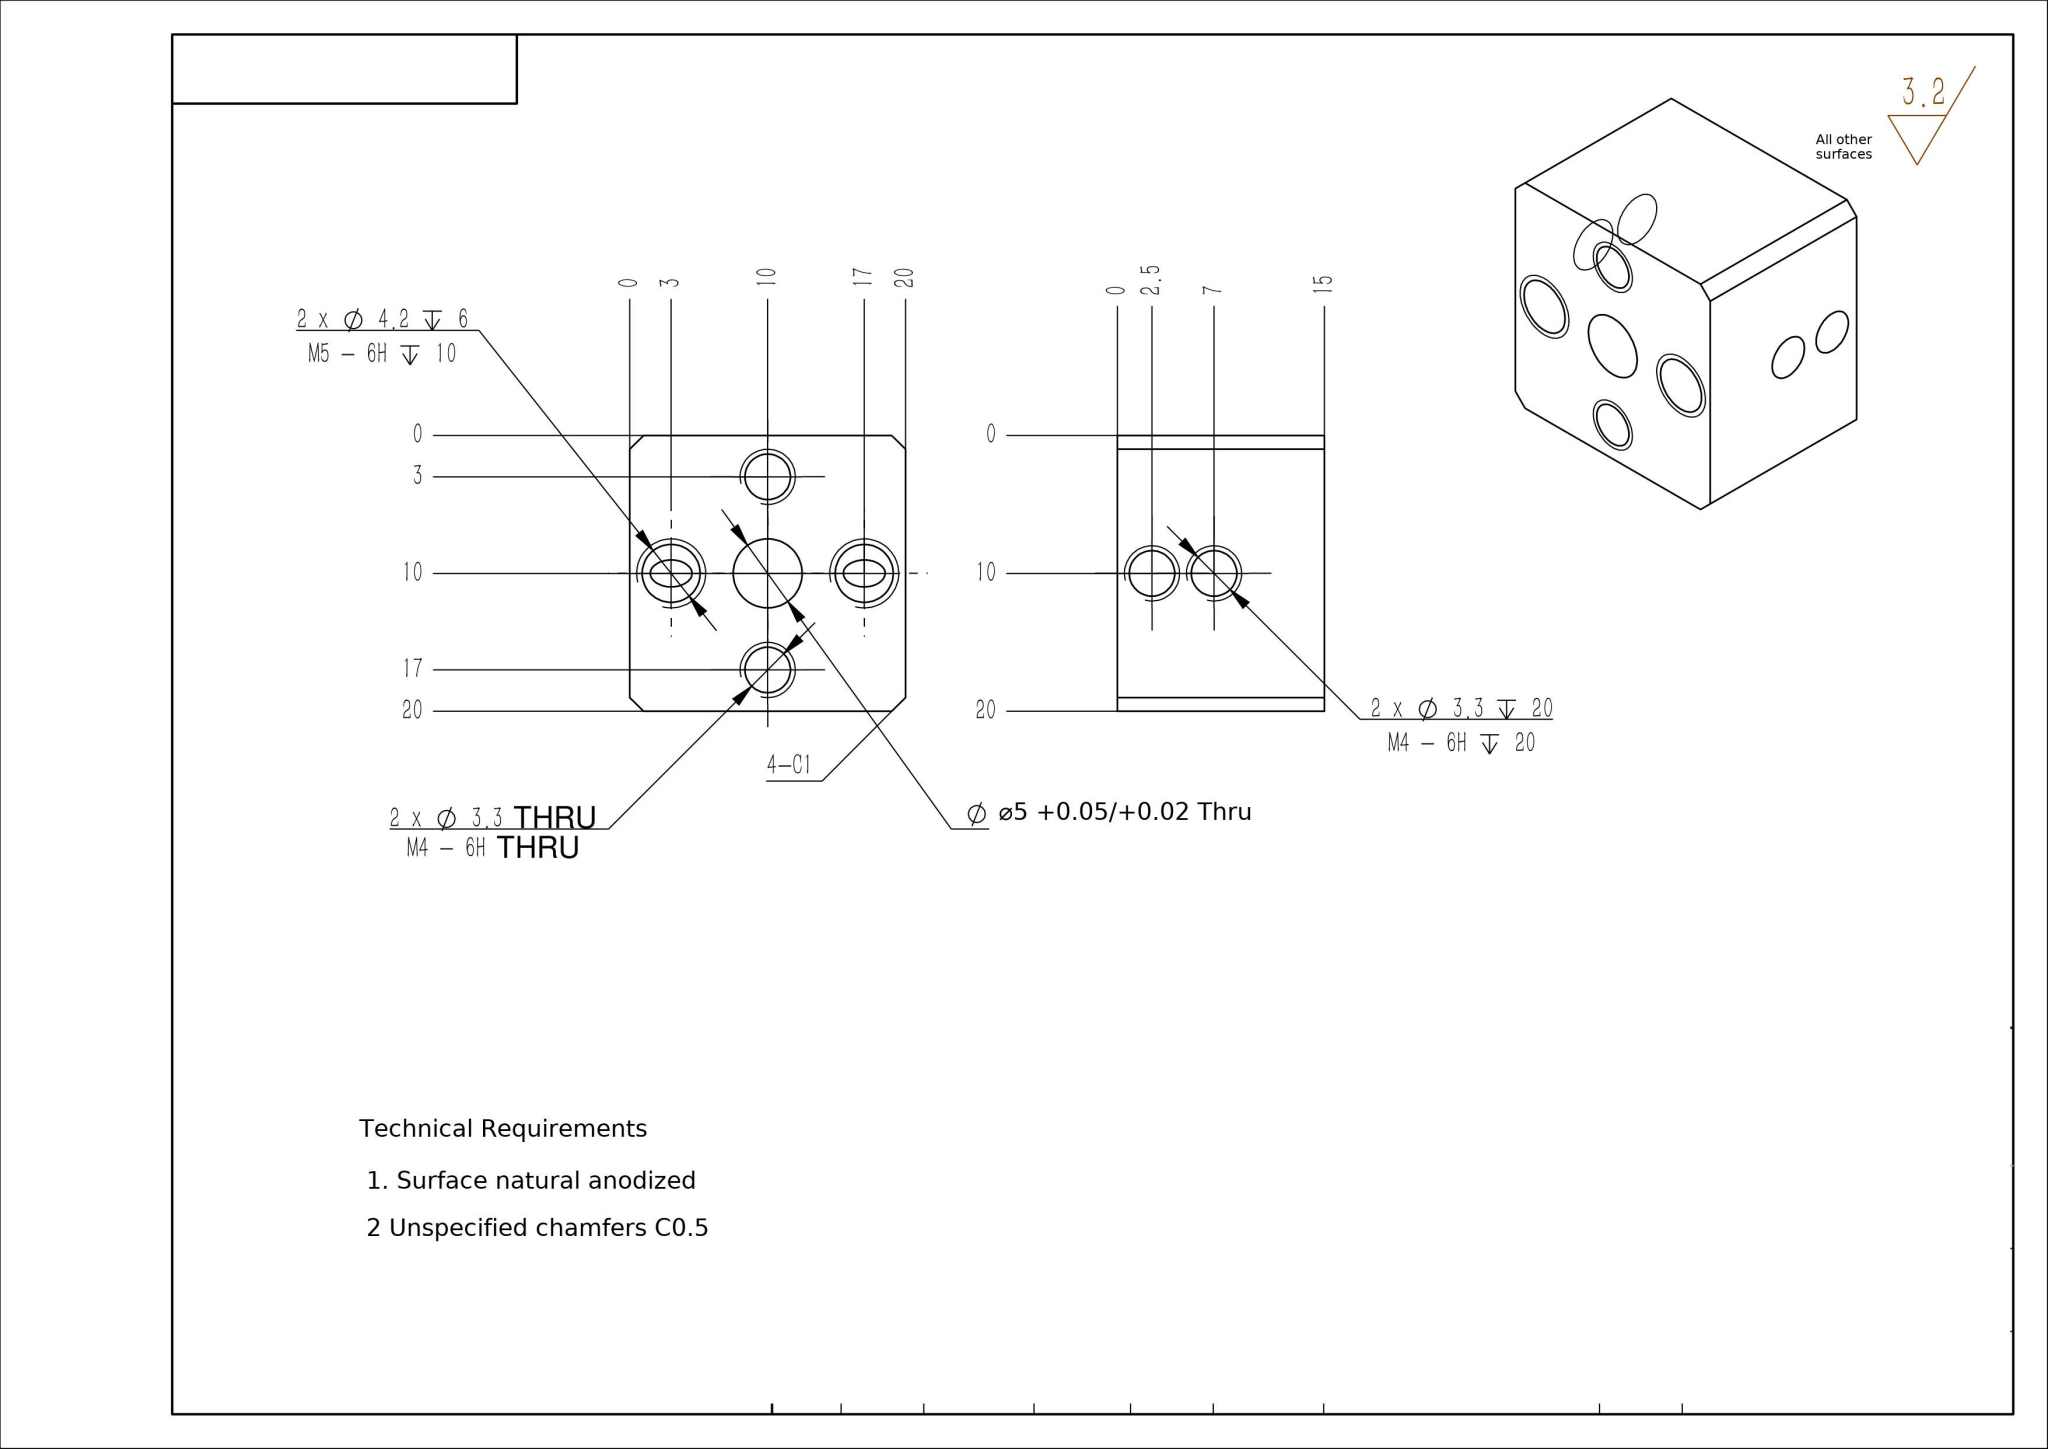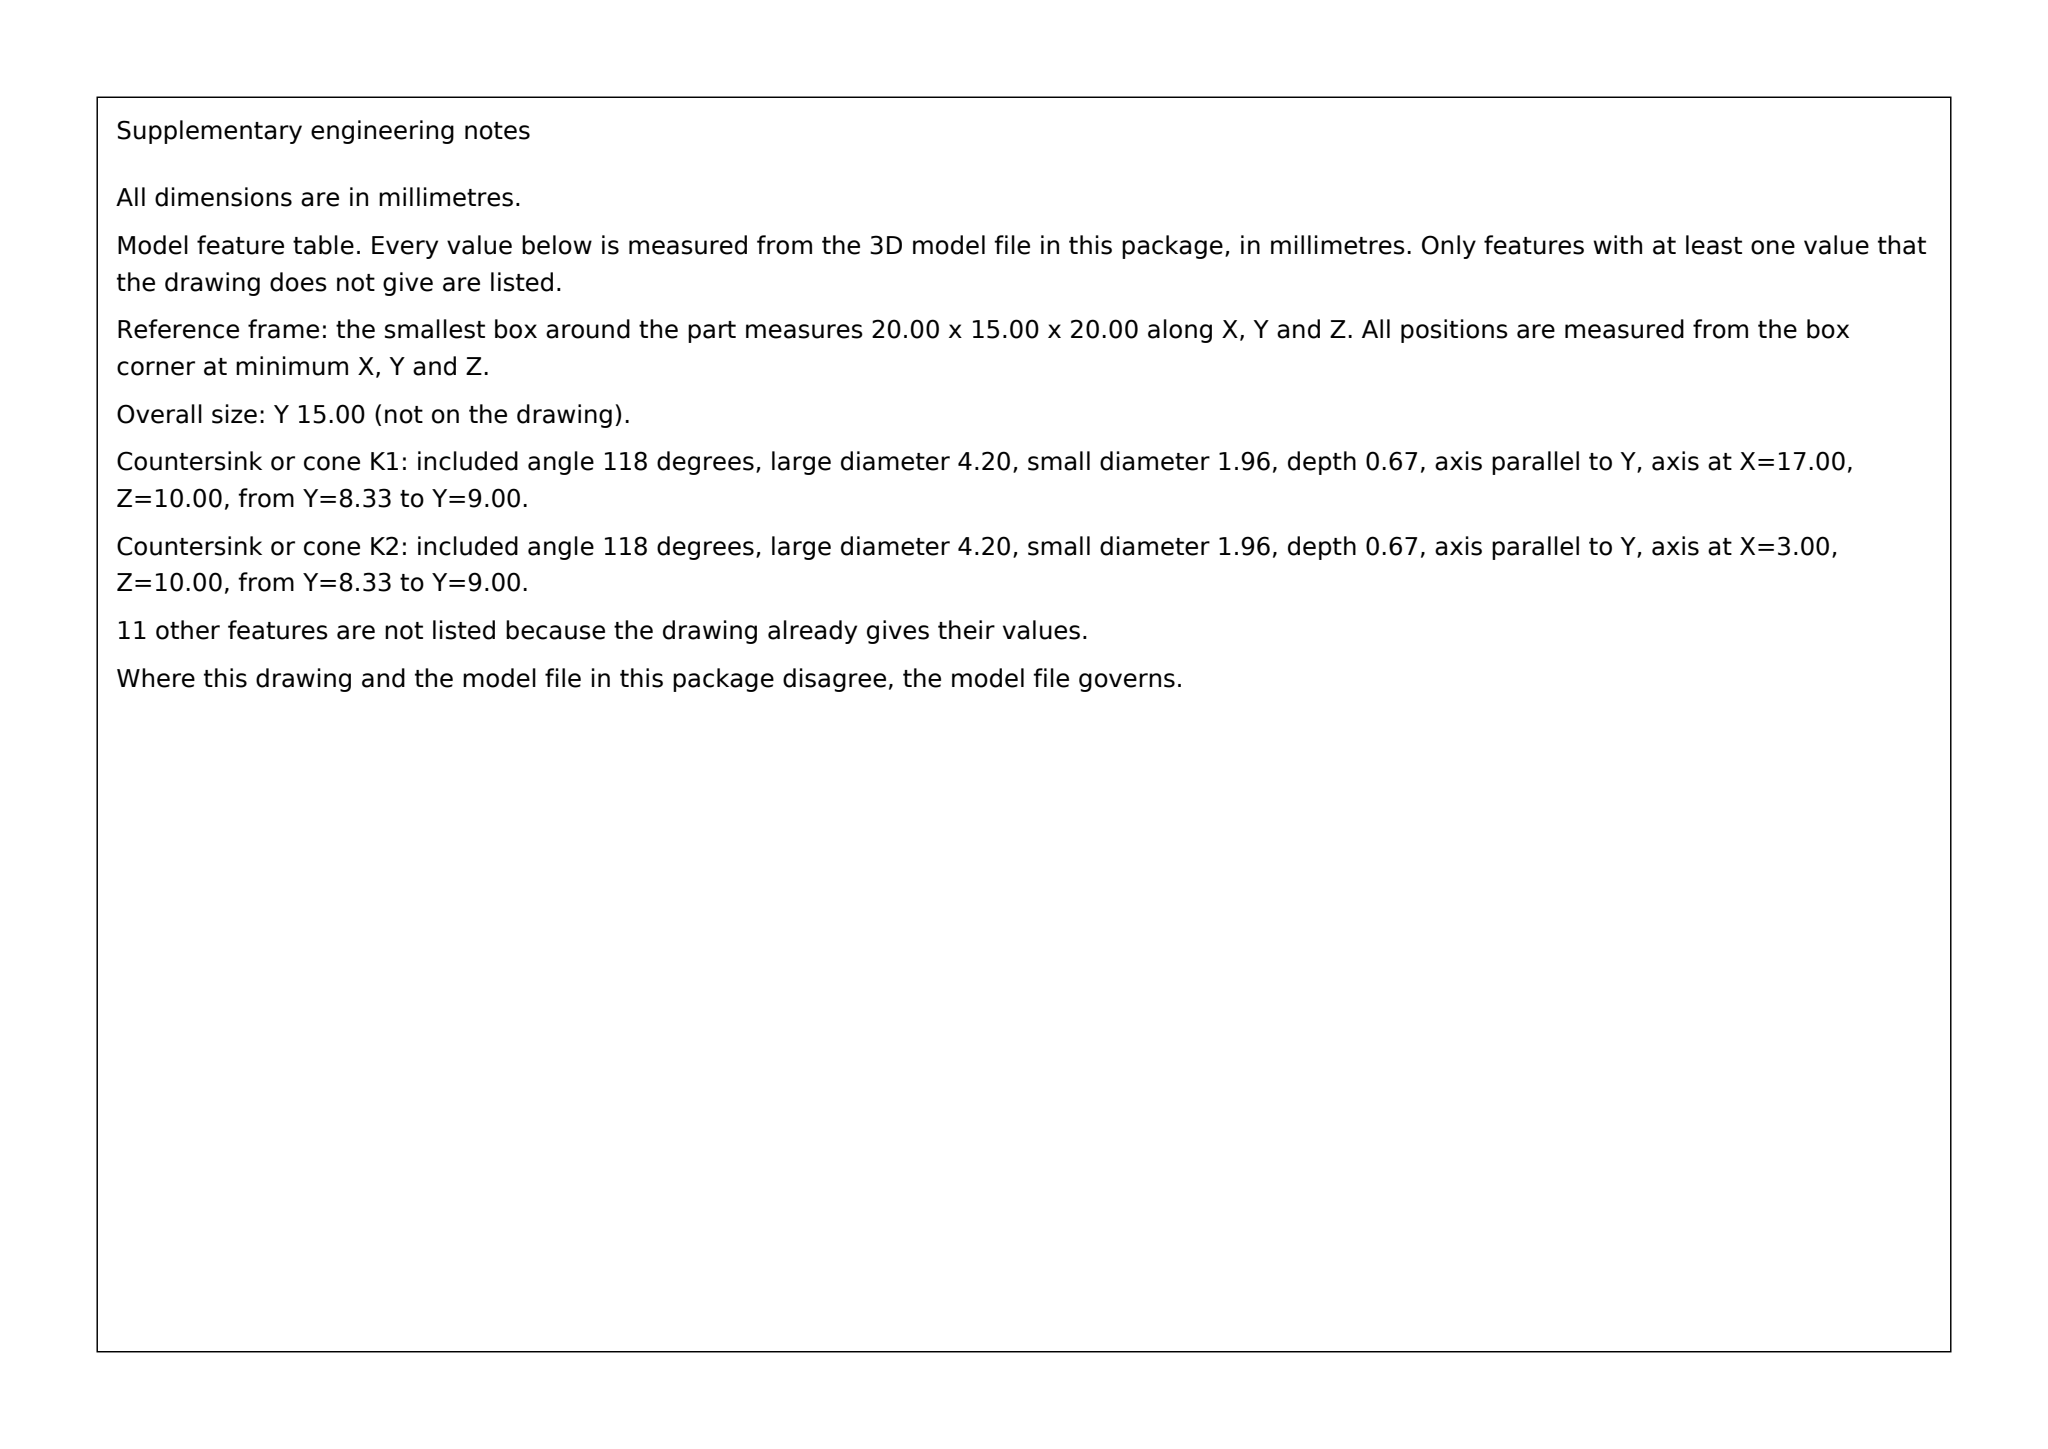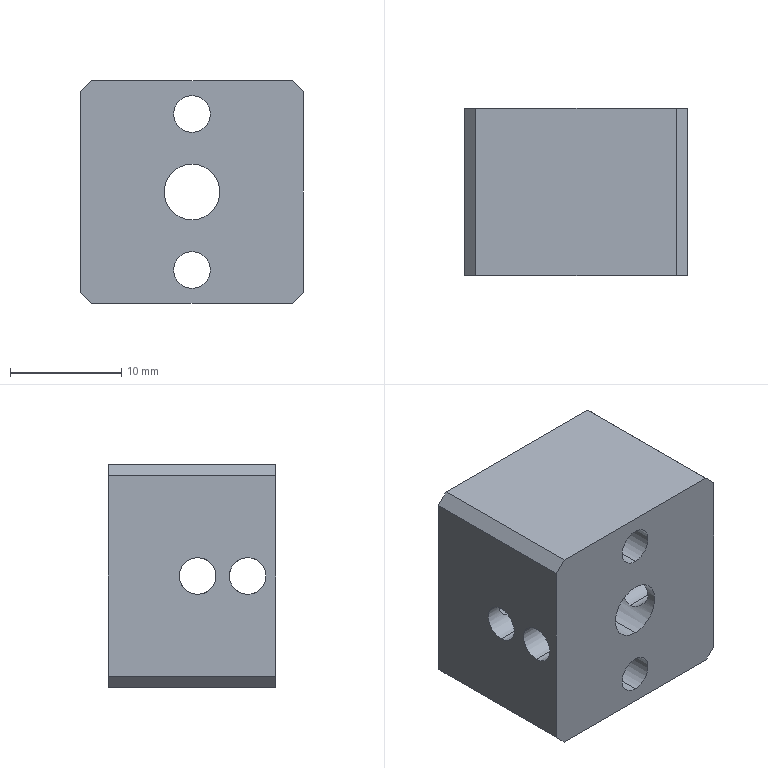Part | SolidWorks | mm | 1 solid | 32 faces | box 20 x 15 x 20 mm | volume 4983 mm3 | cylinder 18 | plane 10 | cone 4 | commonest cylinder face diameters 3.3 x12 4.2 x4 5 x2
build123d program:
from build123d import *

# Parameters (mm, degrees)
SKETCH1_W             = 20
SKETCH1_H             = 20
BOSS_EXTRUDE1_DEPTH   = 15
SKETCH2_R             = 2.5
CUT_EXTRUDE1_DEPTH    = 21.616
M4_TAPPED_HOLE1_D     = 3.3
M4_TAPPED_HOLE2_D     = 3.3
CHAMFER1_SIZE         = 1
M5_TAPPED_HOLE1_D     = 4.2
M5_TAPPED_HOLE1_DEPTH = 6
M5_TAPPED_HOLE1_TIP   = 1.262


with BuildPart() as part:
    # Sketch1 → Boss-Extrude1 (new body)
    with BuildSketch(Plane(origin=(0, 0, 0), x_dir=(1, 0, 0), z_dir=(0, 1, 0))):
        Rectangle(SKETCH1_W, SKETCH1_H)
    extrude(amount=BOSS_EXTRUDE1_DEPTH)

    # Sketch2 → Cut-Extrude1 (cut, through all)
    with BuildSketch(Plane(origin=(0, 15, 0), x_dir=(1, 0, 0), z_dir=(0, 1, 0))):
        with Locations(Location((0, 0, 0), (0, 0, 270))):
            Circle(SKETCH2_R)
    extrude(amount=-CUT_EXTRUDE1_DEPTH, mode=Mode.SUBTRACT)

    # M4 Tapped Hole1 (through all)
    with Locations(Plane.ZY.offset(10)):
        with Locations((0, 7), (0, 2.5)):
            Hole(M4_TAPPED_HOLE1_D / 2)

    # M4 Tapped Hole2 (through all)
    with Locations(Plane(origin=(0, 15, 0), x_dir=(1, 0, 0), z_dir=(0, 1, 0))):
        with Locations((0, 7), (0, -7)):
            Hole(M4_TAPPED_HOLE2_D / 2)

    # Chamfer1
    chamfer1_edges = [part.edges().sort_by_distance(p)[0] for p in [
        (10, 7.5, 10),
        (-10, 7.5, 10),
        (-10, 7.5, -10),
        (10, 7.5, -10),
    ]]
    chamfer(chamfer1_edges, length=CHAMFER1_SIZE)

    # M5 Tapped Hole1
    with Locations(Plane(origin=(0, 15, 0), x_dir=(1, 0, 0), z_dir=(0, 1, 0))):
        with Locations((7, 0), (-7, 0)):
            Hole(M5_TAPPED_HOLE1_D / 2, depth=M5_TAPPED_HOLE1_DEPTH)
            with Locations((0, 0, -(M5_TAPPED_HOLE1_DEPTH + M5_TAPPED_HOLE1_TIP / 2))):  # 118° drill point
                Cone(0, M5_TAPPED_HOLE1_D / 2, M5_TAPPED_HOLE1_TIP, mode=Mode.SUBTRACT)


solid = part.part